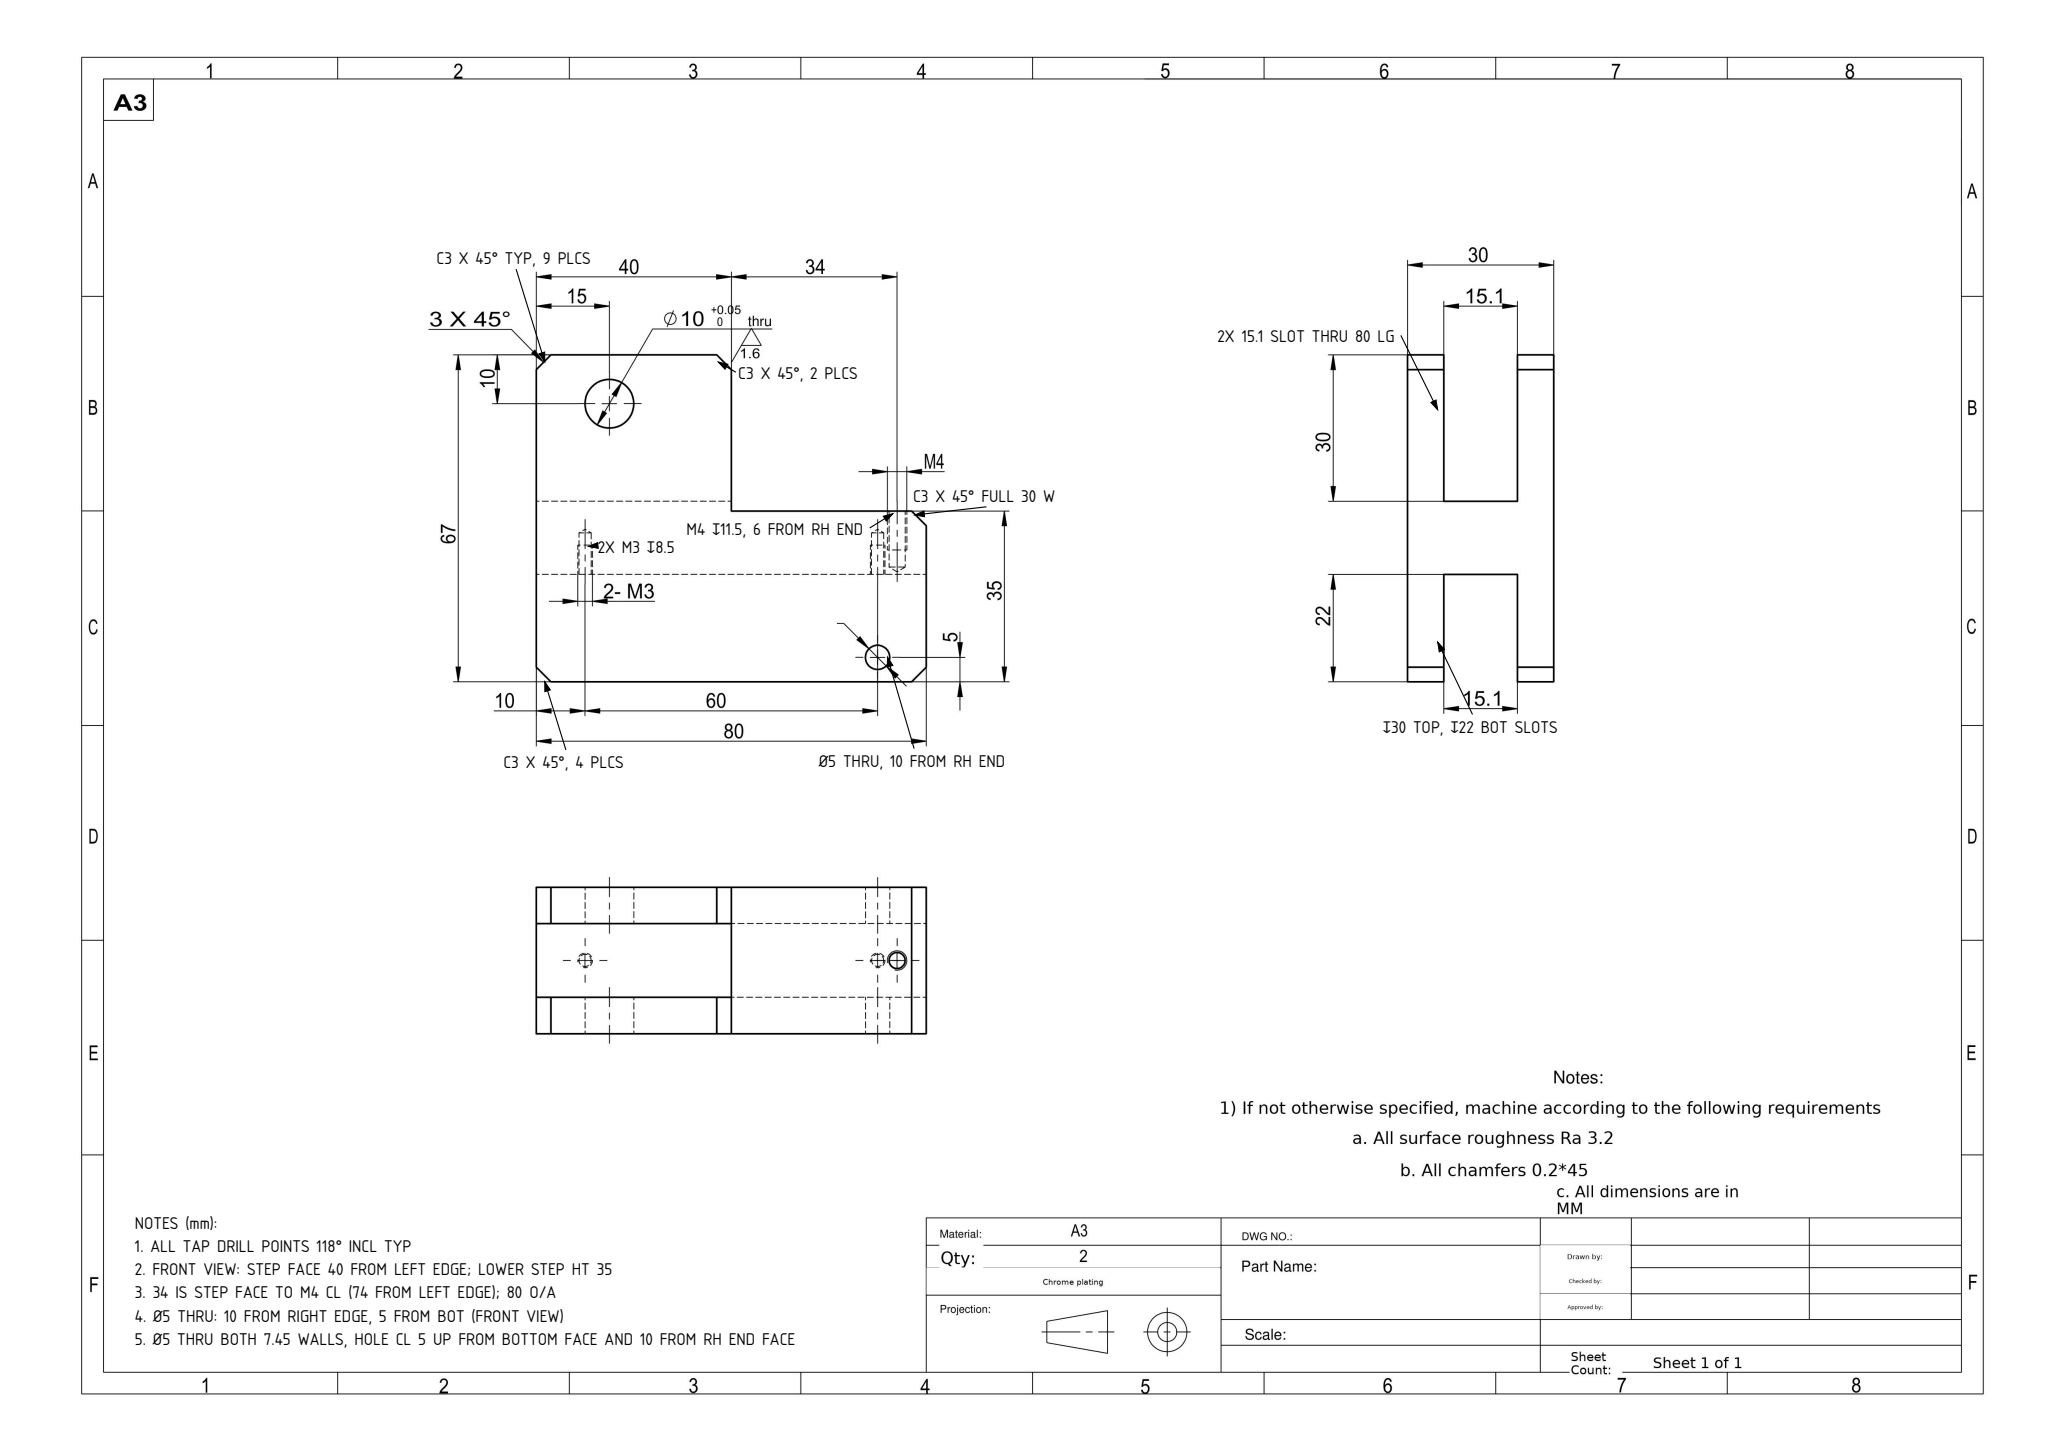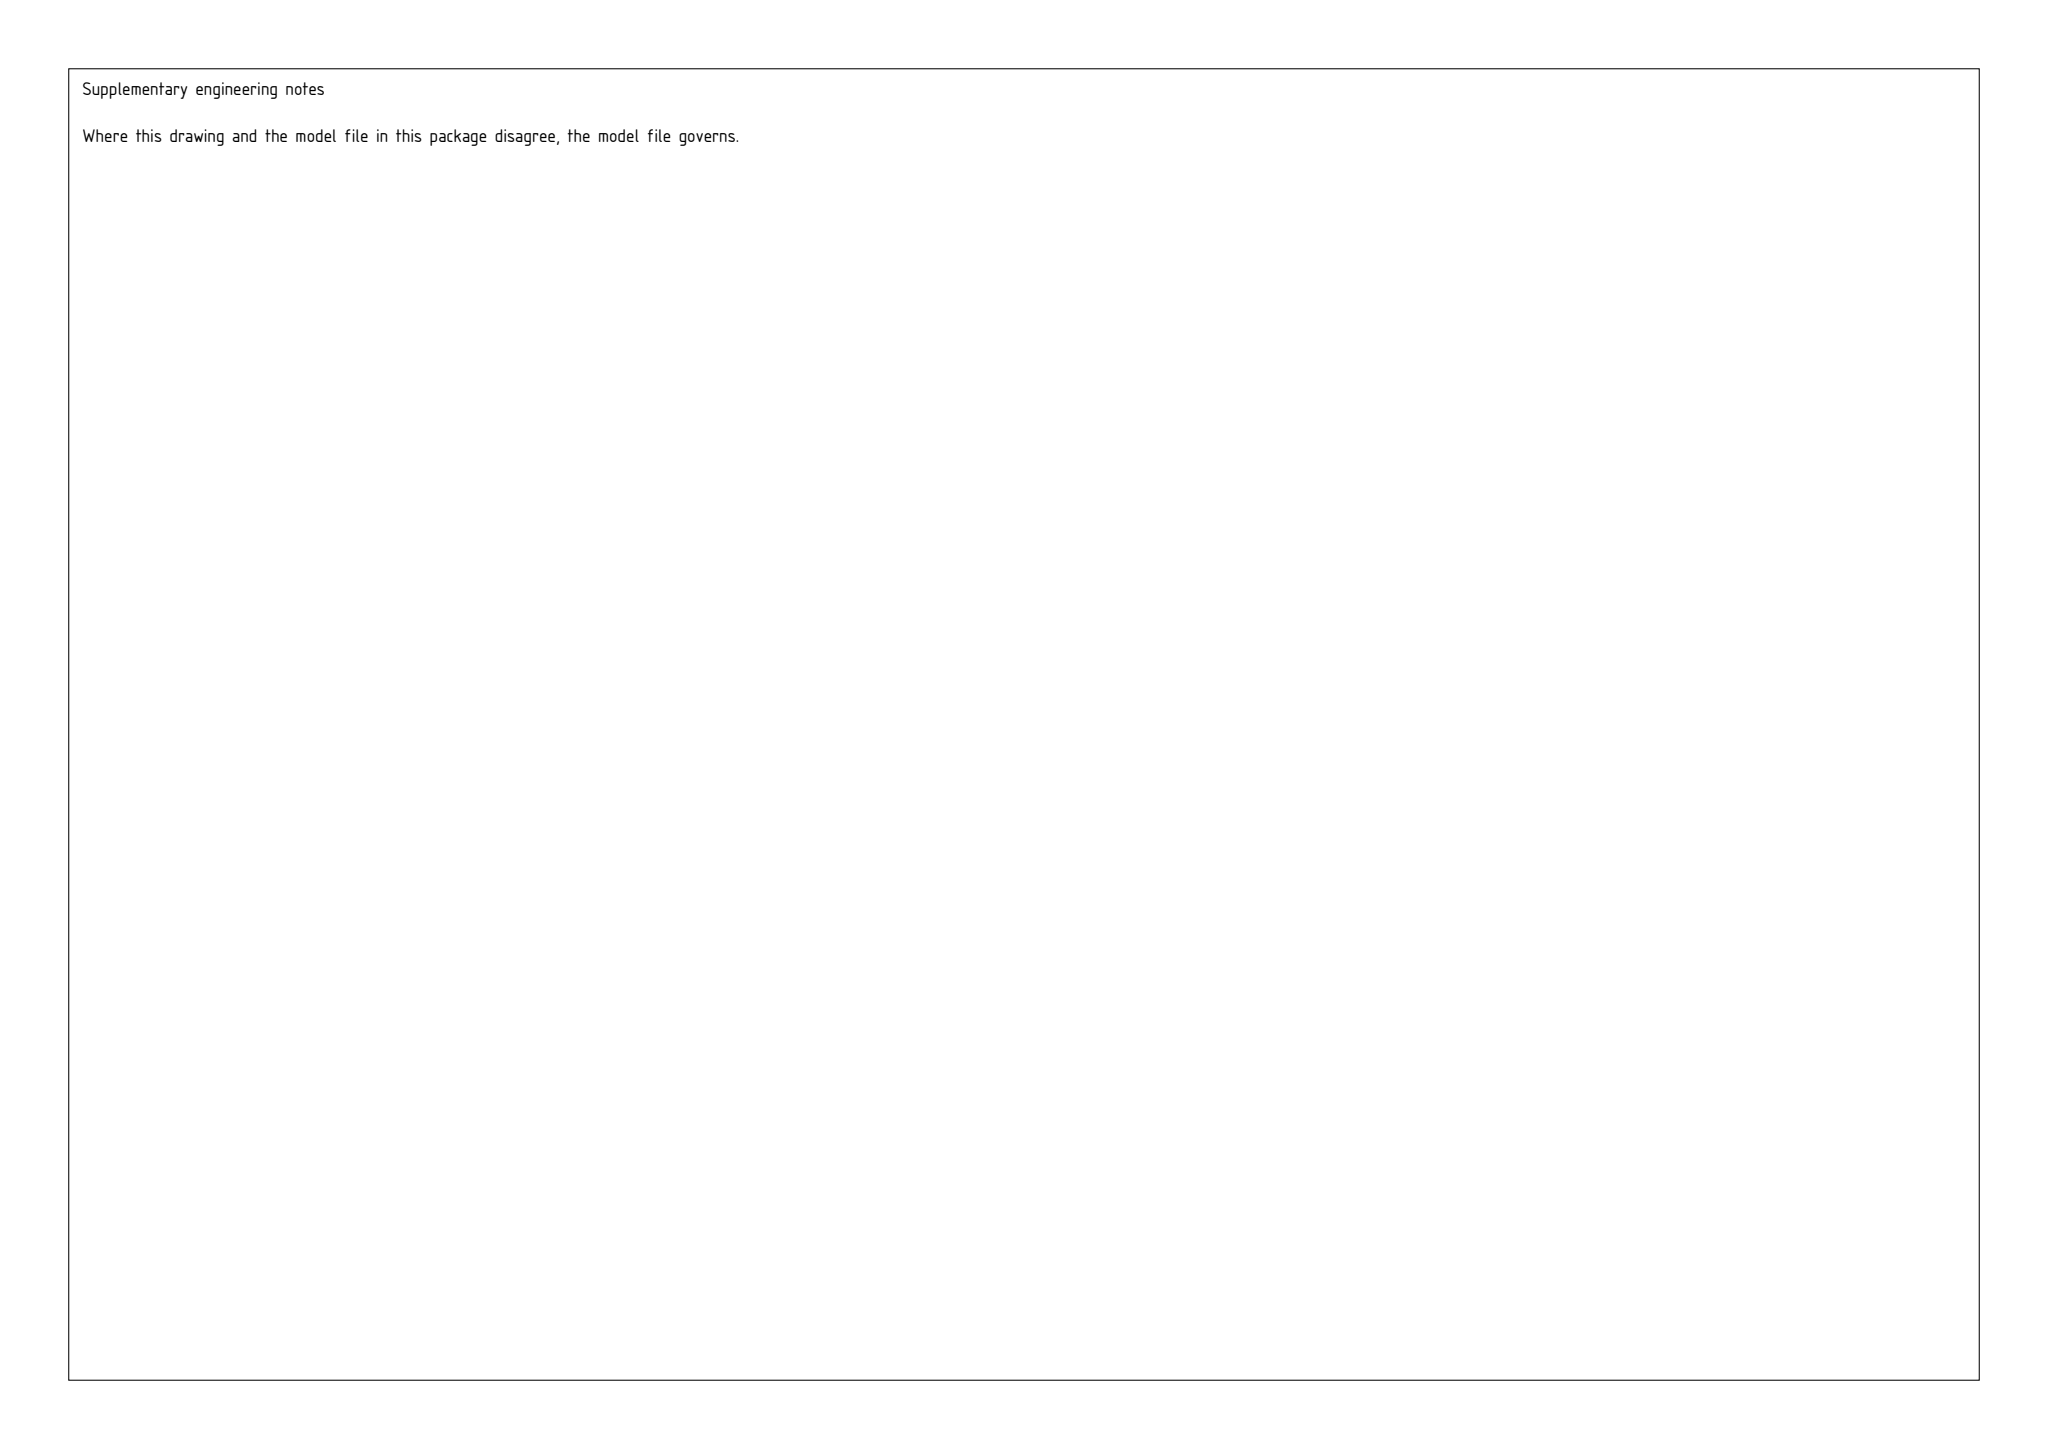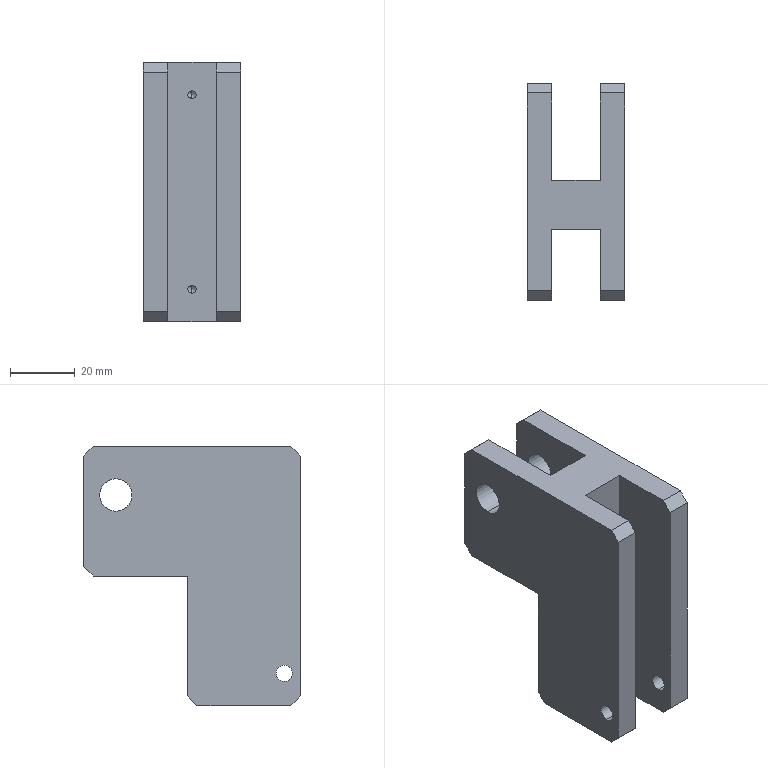Part | SolidWorks | mm | material A3 | 1 solid | 45 faces | box 30 x 67 x 80 mm | volume 75651 mm3 | plane 25 | cylinder 14 | cone 6 | commonest cylinder face diameters 5 x4 2.5 x4 10 x4 3.3 x2
Drawing notes:
BOTH 15.1 SLOTS THRU FULL 80 LG, CTRD ON 30 WIDTH, 7.45 WALL EA SIDE | from the solid: z-planes only at 0/40/80, no slot end faces; x-planes 0/7.45/22.55/30, 7.45+15.1+7.45=30
UPPER SLOT 30 DP EX TOP FACE, LOWER SLOT 22 DP EX BOT FACE | from the solid: y-planes at 37 (67-30) and 22 bounding the 15.1 wide open slots
LOWER RH Ø5 THRU BOTH 7.45 WALLS, CL 10 FROM RH END, 5 UP FROM BOT | from the solid: Ø5 cyl, axis X, y=5, z=10, 4 faces thru both walls
2-M3 DP 8.5 NOT THRU, TAPPED IN SLOT FACE 22 UP FROM BOT | from the solid: Ø2.5 cyl, axis Y, x=15, z=10 & z=70, lg 8.5, 118° pt; y-plane at 22
M4 DP 11.5 NOT THRU IN 35 TOP FACE, CL 6 FROM RH END (74 FROM LH), 15 FROM SIDE | from the solid: Ø3.3 cyl, axis Y, x=15, z=6, lg 11.5, 118° pt; y-plane at 35; bbox z=80
ALL TAP DRILL POINTS 118° INCL TYP | from the solid: cones 118° on Ø3.3 (2) and Ø2.5 (4)
FRONT VIEW: STEP FACE 40 FROM LEFT EDGE; LOWER STEP HT 35 | from the solid: axis plane z=40.0 (vertical step face), y=35.0 (step top face), bbox 80 x 67
34 IS STEP FACE TO M4 CL (74 FROM LEFT EDGE); 80 O/A | from the solid: M4 tap dia 3.3 at z=6.0 -> 74 from opposite end; bbox z=80.0; z=40 step plane
Ø5 THRU: 10 FROM RIGHT EDGE, 5 FROM BOT (FRONT VIEW) | from the solid: cylinder dia 5.0, axis x, pos y=5.0, z=10.0 (=10 from end face z=0, mirrored view)
Ø5 THRU BOTH 7.45 WALLS, HOLE CL 5 UP FROM BOTTOM FACE AND 10 FROM RH END FACE | from the solid: cylinders[dia 5.0, axis x, pos (y=5.0, z=10.0), length 7.45] through the two x-walls bounded by planes x=0/7.45 and x=22.55/30.0
CHAMFER 3 X 45° AT TOP RH CORNER OF 67 HIGH SECTION (AT TOP FACE Y=67 MEETING STEP FACE 40 FROM RH END), BOTH 7.5 WALLS - 2 PLACES | from the solid: inclined_planes 45°: bbox_from [0,64,40] size [7.5,3,3] and bbox_from [22.5,64,40] size [7.5,3,3]
CHAMFER 3 X 45° AT TOP RH CORNER OF 35 HIGH STEP (AT 35 TOP FACE, 0 FROM RH END), FULL 30 WIDTH | from the solid: inclined_planes 45°: bbox_from [0,32,0] size [30,3,3]
CHAMFER 3 X 45° AT BOTTOM LH AND BOTTOM RH CORNERS OF FRONT VIEW (AT BOTTOM FACE Y=0, 0 FROM EACH END), BOTH 7.5 WALLS - 4 PLACES | from the solid: inclined_planes 45°: bbox_from [0,0,0], [22.5,0,0], [0,0,77], [22.5,0,77], each size [7.5,3,3]
ALL CORNER CHAMFERS 3 X 45° TYP, 9 PLACES TOTAL (INCL. TOP LH CORNER 2 PLACES) | from the solid: inclined_planes list: 9 faces, all 45° with 3 x 3 legs
build123d program:
from build123d import *

# Parameters (mm, degrees)
SKETCH1_W               = 30
SKETCH1_H               = 80
BOSS_EXTRUDE1_DEPTH     = 22.5
SKETCH2_W               = 15.1
SKETCH2_H               = 80
CUT_EXTRUDE1_DEPTH      = 30
CUT_EXTRUDE2_DEPTH      = 49.283
CUT_EXTRUDE2_DEPTH_BACK = 49.283
SKETCH4_R               = 5
SKETCH4_W               = 40
SKETCH4_H               = 32
M3_TAPPED_HOLE1_D       = 2.5
M3_TAPPED_HOLE1_DEPTH   = 8.5
M3_TAPPED_HOLE1_TIP     = 0.7511
SKETCH7_W               = 7.45
SKETCH7_H               = 80
BOSS_EXTRUDE2_DEPTH     = 22
CUT_EXTRUDE3_DEPTH      = 62.687
CUT_EXTRUDE3_DEPTH_BACK = 62.687
SKETCH8_R               = 2.5
M4_TAPPED_HOLE1_D       = 3.3
M4_TAPPED_HOLE1_DEPTH   = 11.5
M4_TAPPED_HOLE1_TIP     = 0.9914
CHAMFER1_SIZE           = 3


with BuildPart() as part:
    # Sketch1 → Boss-Extrude1 (new, symmetric)
    with BuildSketch(Plane(origin=(0, 0, 0), x_dir=(1, 0, 0), z_dir=(0, 1, 0))):
        Rectangle(SKETCH1_W, SKETCH1_H)
    extrude(amount=BOSS_EXTRUDE1_DEPTH, both=True)

    # Sketch2 → Cut-Extrude1 (cut)
    with BuildSketch(Plane(origin=(0, 22.5, 0), x_dir=(1, 0, 0), z_dir=(0, 1, 0))):
        Rectangle(SKETCH2_W, SKETCH2_H)
    extrude(amount=-CUT_EXTRUDE1_DEPTH, mode=Mode.SUBTRACT)

    # Sketch4 → Cut-Extrude2 (cut, two sides: drawn at the far end of the back side and taken through both)
    with BuildSketch(Plane(origin=(0, 0, 0), x_dir=(0, 0, -1), z_dir=(1, 0, 0)).offset(-CUT_EXTRUDE2_DEPTH_BACK)):
        with Locations((-25, 12.5)):
            Circle(SKETCH4_R)
        with Locations((20, 6.5)):
            Rectangle(SKETCH4_W, SKETCH4_H)
    extrude(amount=CUT_EXTRUDE2_DEPTH + CUT_EXTRUDE2_DEPTH_BACK, mode=Mode.SUBTRACT)

    # M3 Tapped Hole1
    with Locations(Plane(origin=(0, -22.5, 0), x_dir=(-1, 0, 0), z_dir=(0, -1, 0))):
        with Locations((0, 30), (0, -30)):
            Hole(M3_TAPPED_HOLE1_D / 2, depth=M3_TAPPED_HOLE1_DEPTH)
            with Locations((0, 0, -(M3_TAPPED_HOLE1_DEPTH + M3_TAPPED_HOLE1_TIP / 2))):  # 118° drill point
                Cone(0, M3_TAPPED_HOLE1_D / 2, M3_TAPPED_HOLE1_TIP, mode=Mode.SUBTRACT)

    # Sketch7 → Boss-Extrude2 (add)
    with BuildSketch(Plane.XZ.offset(22.5)):
        with Locations((-11.275, 0)):
            Rectangle(SKETCH7_W, SKETCH7_H)
        with Locations((11.275, 0)):
            Rectangle(SKETCH7_W, SKETCH7_H)
    extrude(amount=BOSS_EXTRUDE2_DEPTH)

    # Sketch8 → Cut-Extrude3 (cut, two sides: drawn at the far end of the back side and taken through both)
    with BuildSketch(Plane(origin=(0, 0, 0), x_dir=(0, 0, -1), z_dir=(1, 0, 0)).offset(-CUT_EXTRUDE3_DEPTH_BACK)):
        with Locations((30, -39.5)):
            Circle(SKETCH8_R)
    extrude(amount=CUT_EXTRUDE3_DEPTH + CUT_EXTRUDE3_DEPTH_BACK, mode=Mode.SUBTRACT)

    # M4 Tapped Hole1
    with Locations(Plane(origin=(0, -9.5, 0), x_dir=(1, 0, 0), z_dir=(0, 1, 0))):
        with Locations((0, 34)):
            Hole(M4_TAPPED_HOLE1_D / 2, depth=M4_TAPPED_HOLE1_DEPTH)
            with Locations((0, 0, -(M4_TAPPED_HOLE1_DEPTH + M4_TAPPED_HOLE1_TIP / 2))):  # 118° drill point
                Cone(0, M4_TAPPED_HOLE1_D / 2, M4_TAPPED_HOLE1_TIP, mode=Mode.SUBTRACT)

    # Chamfer1
    chamfer1_edges = [part.edges().sort_by_distance(p)[0] for p in [
        (-11.275, 22.5, 40),
        (11.275, 22.5, 40),
        (-11.275, 22.5, 0),
        (11.275, 22.5, 0),
        (0, -9.5, -40),
        (-11.275, -44.5, -40),
        (-11.275, -44.5, 40),
        (11.275, -44.5, 40),
        (11.275, -44.5, -40),
    ]]
    chamfer(chamfer1_edges, length=CHAMFER1_SIZE)


solid = part.part